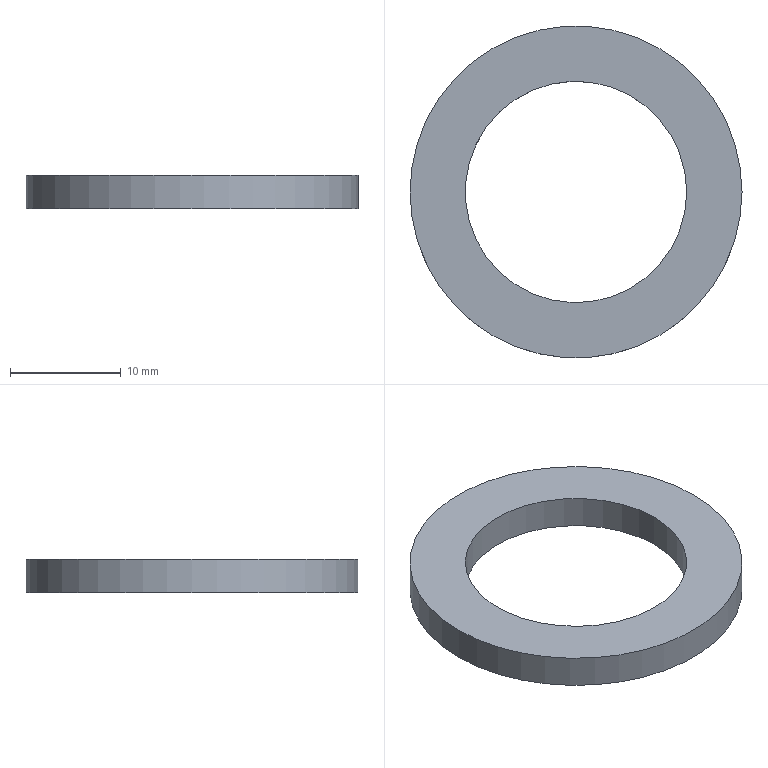Component | NX | WASHER_2 | 1 solid | 4 faces | box 30 x 30 x 3 mm | volume 1178 mm3 | cylinder 2 | plane 2 | commonest cylinder face diameters 30 x1 20 x1
STEP:
#1=CARTESIAN_POINT('',(0.,0.,0.));
#2=DIRECTION('',(0.,0.,1.));
#3=DIRECTION('',(1.,0.,0.));
#4=AXIS2_PLACEMENT_3D('',#1,#2,#3);
#5=CARTESIAN_POINT('',(1475.132,1212.,801.574));
#6=VERTEX_POINT('',#5);
#7=CARTESIAN_POINT('',(1460.132,1212.,801.574));
#8=DIRECTION('',(0.,0.,1.));
#9=DIRECTION('',(1.,0.,0.));
#10=AXIS2_PLACEMENT_3D('',#7,#8,#9);
#11=CIRCLE('',#10,15.);
#12=CARTESIAN_POINT('',(1460.132,1212.,801.574));
#13=DIRECTION('',(0.,0.,1.));
#14=DIRECTION('',(1.,0.,0.));
#15=AXIS2_PLACEMENT_3D('',#12,#13,#14);
#16=CYLINDRICAL_SURFACE('',#15,15.);
#17=CARTESIAN_POINT('',(0.,0.));
#18=DIRECTION('',(1.,0.));
#19=VECTOR('',#18,1.);
#20=LINE('',#17,#19);
#21=(GEOMETRIC_REPRESENTATION_CONTEXT(2)PARAMETRIC_REPRESENTATION_CONTEXT()REPRESENTATION_CONTEXT('',''));
#22=DEFINITIONAL_REPRESENTATION('',(#20),#21);
#23=PCURVE('',#16,#22);
#24=CARTESIAN_POINT('',(1460.132,1212.,801.574));
#25=DIRECTION('',(0.,0.,1.));
#26=DIRECTION('',(1.,0.,0.));
#27=AXIS2_PLACEMENT_3D('',#24,#25,#26);
#28=PLANE('',#27);
#29=CARTESIAN_POINT('',(0.,0.));
#30=DIRECTION('',(1.,0.));
#31=AXIS2_PLACEMENT_2D('',#29,#30);
#32=CIRCLE('',#31,15.);
#33=(GEOMETRIC_REPRESENTATION_CONTEXT(2)PARAMETRIC_REPRESENTATION_CONTEXT()REPRESENTATION_CONTEXT('',''));
#34=DEFINITIONAL_REPRESENTATION('',(#32),#33);
#35=PCURVE('',#28,#34);
#36=SURFACE_CURVE('',#11,(#23,#35),.PCURVE_S1.);
#37=EDGE_CURVE('',#6,#6,#36,.T.);
#38=ORIENTED_EDGE('',*,*,#37,.T.);
#39=CARTESIAN_POINT('',(1475.132,1212.,804.574));
#40=VERTEX_POINT('',#39);
#41=CARTESIAN_POINT('',(1475.132,1212.,801.574));
#42=CARTESIAN_POINT('',(1475.132,1212.,804.574));
#43=B_SPLINE_CURVE_WITH_KNOTS('',1,(#41,#42),.UNSPECIFIED.,.F.,.F.,(2,2),(0.,3.),.PIECEWISE_BEZIER_KNOTS.);
#44=CARTESIAN_POINT('',(6.283,0.));
#45=DIRECTION('',(0.,1.));
#46=VECTOR('',#45,1.);
#47=LINE('',#44,#46);
#48=(GEOMETRIC_REPRESENTATION_CONTEXT(2)PARAMETRIC_REPRESENTATION_CONTEXT()REPRESENTATION_CONTEXT('',''));
#49=DEFINITIONAL_REPRESENTATION('',(#47),#48);
#50=PCURVE('',#16,#49);
#51=CARTESIAN_POINT('',(0.,0.));
#52=DIRECTION('',(0.,1.));
#53=VECTOR('',#52,1.);
#54=LINE('',#51,#53);
#55=(GEOMETRIC_REPRESENTATION_CONTEXT(2)PARAMETRIC_REPRESENTATION_CONTEXT()REPRESENTATION_CONTEXT('',''));
#56=DEFINITIONAL_REPRESENTATION('',(#54),#55);
#57=PCURVE('',#16,#56);
#58=SEAM_CURVE('',#43,(#50,#57),.PCURVE_S1.);
#59=EDGE_CURVE('',#6,#40,#58,.T.);
#60=ORIENTED_EDGE('',*,*,#59,.T.);
#61=CARTESIAN_POINT('',(1460.132,1212.,804.574));
#62=DIRECTION('',(0.,0.,1.));
#63=DIRECTION('',(1.,0.,0.));
#64=AXIS2_PLACEMENT_3D('',#61,#62,#63);
#65=CIRCLE('',#64,15.);
#66=CARTESIAN_POINT('',(0.,3.));
#67=DIRECTION('',(1.,0.));
#68=VECTOR('',#67,1.);
#69=LINE('',#66,#68);
#70=(GEOMETRIC_REPRESENTATION_CONTEXT(2)PARAMETRIC_REPRESENTATION_CONTEXT()REPRESENTATION_CONTEXT('',''));
#71=DEFINITIONAL_REPRESENTATION('',(#69),#70);
#72=PCURVE('',#16,#71);
#73=CARTESIAN_POINT('',(1460.132,1212.,804.574));
#74=DIRECTION('',(0.,0.,1.));
#75=DIRECTION('',(1.,0.,0.));
#76=AXIS2_PLACEMENT_3D('',#73,#74,#75);
#77=PLANE('',#76);
#78=CARTESIAN_POINT('',(0.,0.));
#79=DIRECTION('',(1.,0.));
#80=AXIS2_PLACEMENT_2D('',#78,#79);
#81=CIRCLE('',#80,15.);
#82=(GEOMETRIC_REPRESENTATION_CONTEXT(2)PARAMETRIC_REPRESENTATION_CONTEXT()REPRESENTATION_CONTEXT('',''));
#83=DEFINITIONAL_REPRESENTATION('',(#81),#82);
#84=PCURVE('',#77,#83);
#85=SURFACE_CURVE('',#65,(#72,#84),.PCURVE_S1.);
#86=EDGE_CURVE('',#40,#40,#85,.T.);
#87=ORIENTED_EDGE('',*,*,#86,.F.);
#88=ORIENTED_EDGE('',*,*,#59,.F.);
#89=EDGE_LOOP('',(#38,#60,#87,#88));
#90=FACE_BOUND('',#89,.T.);
#91=ADVANCED_FACE('',(#90),#16,.T.);
#92=CARTESIAN_POINT('',(1470.132,1212.,801.574));
#93=VERTEX_POINT('',#92);
#94=CARTESIAN_POINT('',(1460.132,1212.,801.574));
#95=DIRECTION('',(0.,0.,1.));
#96=DIRECTION('',(1.,0.,0.));
#97=AXIS2_PLACEMENT_3D('',#94,#95,#96);
#98=CIRCLE('',#97,10.);
#99=CARTESIAN_POINT('',(1460.132,1212.,801.574));
#100=DIRECTION('',(0.,0.,1.));
#101=DIRECTION('',(1.,0.,0.));
#102=AXIS2_PLACEMENT_3D('',#99,#100,#101);
#103=CYLINDRICAL_SURFACE('',#102,10.);
#104=CARTESIAN_POINT('',(0.,0.));
#105=DIRECTION('',(1.,0.));
#106=VECTOR('',#105,1.);
#107=LINE('',#104,#106);
#108=(GEOMETRIC_REPRESENTATION_CONTEXT(2)PARAMETRIC_REPRESENTATION_CONTEXT()REPRESENTATION_CONTEXT('',''));
#109=DEFINITIONAL_REPRESENTATION('',(#107),#108);
#110=PCURVE('',#103,#109);
#111=CARTESIAN_POINT('',(0.,0.));
#112=DIRECTION('',(1.,0.));
#113=AXIS2_PLACEMENT_2D('',#111,#112);
#114=CIRCLE('',#113,10.);
#115=(GEOMETRIC_REPRESENTATION_CONTEXT(2)PARAMETRIC_REPRESENTATION_CONTEXT()REPRESENTATION_CONTEXT('',''));
#116=DEFINITIONAL_REPRESENTATION('',(#114),#115);
#117=PCURVE('',#28,#116);
#118=SURFACE_CURVE('',#98,(#110,#117),.PCURVE_S1.);
#119=EDGE_CURVE('',#93,#93,#118,.T.);
#120=ORIENTED_EDGE('',*,*,#119,.T.);
#121=CARTESIAN_POINT('',(1470.132,1212.,804.574));
#122=VERTEX_POINT('',#121);
#123=CARTESIAN_POINT('',(1470.132,1212.,801.574));
#124=CARTESIAN_POINT('',(1470.132,1212.,804.574));
#125=B_SPLINE_CURVE_WITH_KNOTS('',1,(#123,#124),.UNSPECIFIED.,.F.,.F.,(2,2),(0.,3.),.PIECEWISE_BEZIER_KNOTS.);
#126=CARTESIAN_POINT('',(6.283,0.));
#127=DIRECTION('',(0.,1.));
#128=VECTOR('',#127,1.);
#129=LINE('',#126,#128);
#130=(GEOMETRIC_REPRESENTATION_CONTEXT(2)PARAMETRIC_REPRESENTATION_CONTEXT()REPRESENTATION_CONTEXT('',''));
#131=DEFINITIONAL_REPRESENTATION('',(#129),#130);
#132=PCURVE('',#103,#131);
#133=CARTESIAN_POINT('',(0.,0.));
#134=DIRECTION('',(0.,1.));
#135=VECTOR('',#134,1.);
#136=LINE('',#133,#135);
#137=(GEOMETRIC_REPRESENTATION_CONTEXT(2)PARAMETRIC_REPRESENTATION_CONTEXT()REPRESENTATION_CONTEXT('',''));
#138=DEFINITIONAL_REPRESENTATION('',(#136),#137);
#139=PCURVE('',#103,#138);
#140=SEAM_CURVE('',#125,(#132,#139),.PCURVE_S1.);
#141=EDGE_CURVE('',#93,#122,#140,.T.);
#142=ORIENTED_EDGE('',*,*,#141,.T.);
#143=CARTESIAN_POINT('',(1460.132,1212.,804.574));
#144=DIRECTION('',(0.,0.,1.));
#145=DIRECTION('',(1.,0.,0.));
#146=AXIS2_PLACEMENT_3D('',#143,#144,#145);
#147=CIRCLE('',#146,10.);
#148=CARTESIAN_POINT('',(0.,3.));
#149=DIRECTION('',(1.,0.));
#150=VECTOR('',#149,1.);
#151=LINE('',#148,#150);
#152=(GEOMETRIC_REPRESENTATION_CONTEXT(2)PARAMETRIC_REPRESENTATION_CONTEXT()REPRESENTATION_CONTEXT('',''));
#153=DEFINITIONAL_REPRESENTATION('',(#151),#152);
#154=PCURVE('',#103,#153);
#155=CARTESIAN_POINT('',(0.,0.));
#156=DIRECTION('',(1.,0.));
#157=AXIS2_PLACEMENT_2D('',#155,#156);
#158=CIRCLE('',#157,10.);
#159=(GEOMETRIC_REPRESENTATION_CONTEXT(2)PARAMETRIC_REPRESENTATION_CONTEXT()REPRESENTATION_CONTEXT('',''));
#160=DEFINITIONAL_REPRESENTATION('',(#158),#159);
#161=PCURVE('',#77,#160);
#162=SURFACE_CURVE('',#147,(#154,#161),.PCURVE_S1.);
#163=EDGE_CURVE('',#122,#122,#162,.T.);
#164=ORIENTED_EDGE('',*,*,#163,.F.);
#165=ORIENTED_EDGE('',*,*,#141,.F.);
#166=EDGE_LOOP('',(#120,#142,#164,#165));
#167=FACE_BOUND('',#166,.F.);
#168=ADVANCED_FACE('',(#167),#103,.F.);
#169=ORIENTED_EDGE('',*,*,#37,.F.);
#170=EDGE_LOOP('',(#169));
#171=FACE_BOUND('',#170,.T.);
#172=ORIENTED_EDGE('',*,*,#119,.T.);
#173=EDGE_LOOP('',(#172));
#174=FACE_BOUND('',#173,.T.);
#175=ADVANCED_FACE('',(#171,#174),#28,.F.);
#176=ORIENTED_EDGE('',*,*,#86,.T.);
#177=EDGE_LOOP('',(#176));
#178=FACE_BOUND('',#177,.T.);
#179=ORIENTED_EDGE('',*,*,#163,.F.);
#180=EDGE_LOOP('',(#179));
#181=FACE_BOUND('',#180,.T.);
#182=ADVANCED_FACE('',(#178,#181),#77,.T.);
#183=CLOSED_SHELL('',(#91,#168,#175,#182));
#184=MANIFOLD_SOLID_BREP('',#183);
#185=(LENGTH_UNIT()NAMED_UNIT(*)SI_UNIT(.MILLI.,.METRE.));
#186=UNCERTAINTY_MEASURE_WITH_UNIT(LENGTH_MEASURE(0.00001),#185,'','');
#187=(NAMED_UNIT(*)PLANE_ANGLE_UNIT()SI_UNIT($,.RADIAN.));
#188=(NAMED_UNIT(*)SI_UNIT($,.STERADIAN.)SOLID_ANGLE_UNIT());
#189=(GEOMETRIC_REPRESENTATION_CONTEXT(3)GLOBAL_UNCERTAINTY_ASSIGNED_CONTEXT((#186))GLOBAL_UNIT_ASSIGNED_CONTEXT((#185,#187,#188))REPRESENTATION_CONTEXT('',''));
#190=ADVANCED_BREP_SHAPE_REPRESENTATION('',(#4,#184),#189);